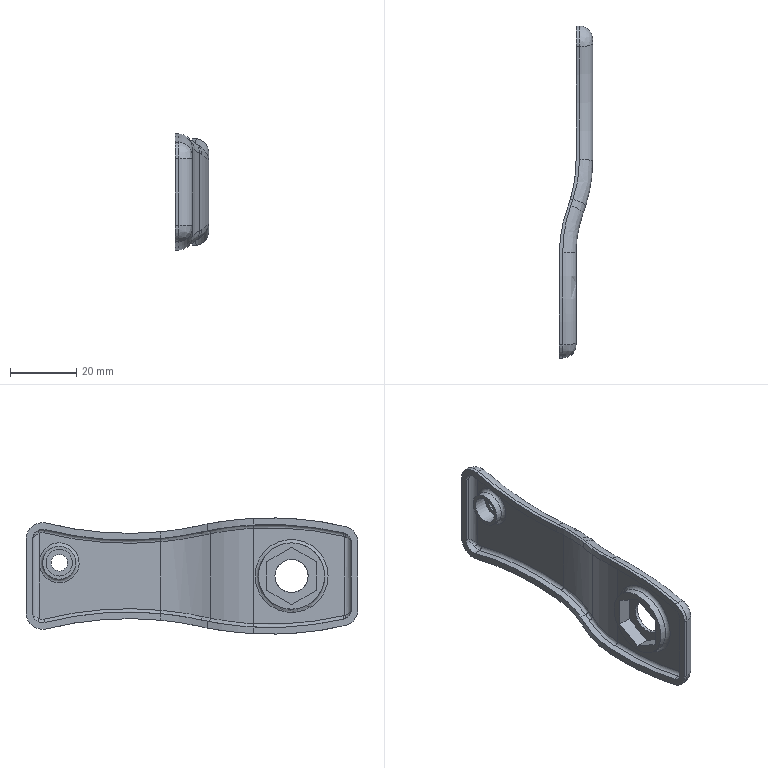Component | NX | HANDLE | 1 solid | 87 faces | volume 6920 mm3 | cylinder 33 | plane 20 | spline 20 | torus 14 | commonest cylinder face diameters 10 x6 80 x4 200 x4 6 x4 8 x3 204 x2 196 x2 4 x2